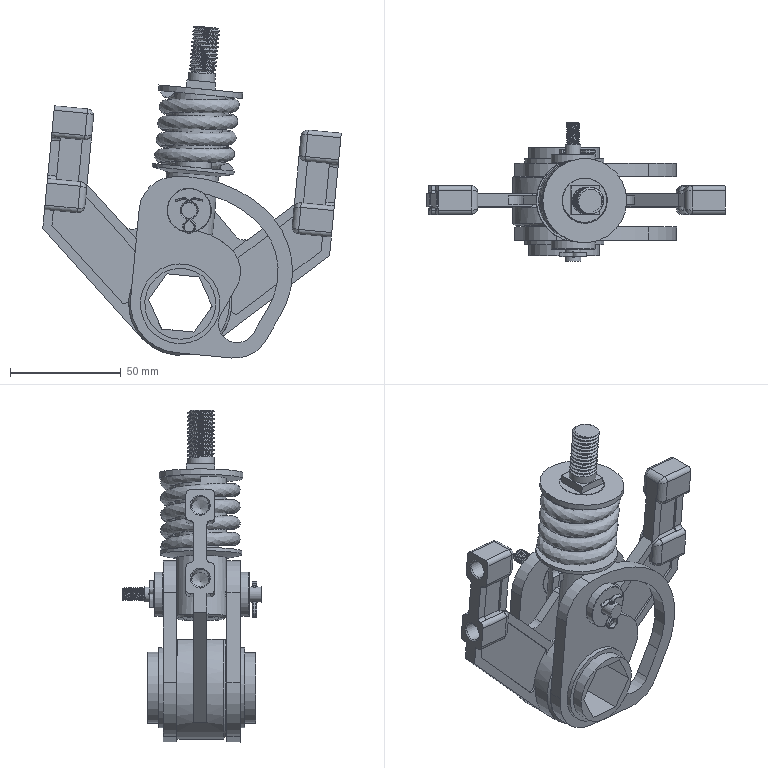Assembly | NX | mm | 14 component files | 14 solids | 384 faces | box 134.7 x 62.5 x 149.86 mm | volume 133468 mm3 | plane 178 | cylinder 147 | spline 30 | cone 23 | torus 6 | commonest cylinder face diameters 6 x25 4 x24 12 x12 7 x12 32 x8 3 x8 17 x6 10 x6
Bill of materials:
unnamed part 1 | 2 |  | Thick annular ring (spacer/washer-like) with a central through bore and small chamfers on the outer edges.
unnamed part 2 | 1 |  | Flat plate with a rounded, roughly D/teardrop outline, a large curved hook-shaped through slot, and a hexagonal feature with stepped cylindrical collars protruding on both faces.
unnamed part 3 | 1 |  | Flanged cylindrical sleeve with a thin wide flange, a through bore, a radial cross hole, and an axial slot running from the open end that ends in a rounded keyhole-like shape.
unnamed part 4 | 2 |  | Flat annular washer-like ring with a central through hole, thinner relative to its diameter than unnamed part 1, with small edge rounds or chamfers.
unnamed part 5 | 1 |  | Flanged plain bushing: cylindrical sleeve with a thin outer flange at one end, a through bore, an annular recess or counterbore on the flange face, and a chamfer at the other end.
unnamed part 6 | 1 |  | Bent strip or wire form clip: a closed circular eye, two parallel straight legs side by side, and leg ends that bend outward in opposite directions at an angle.
unnamed part 7 | 1 |  | Solid cylindrical pin with an external thread at one end and two radial cross holes, one near each end.
unnamed part 8 | 1 |  | Open helical coil spring of round wire with about four to five active turns and cut-off flat ends.
unnamed part 9 | 1 |  | Flat plate with a rounded, roughly D/teardrop outline, a large curved hook-shaped through slot, and a hexagonal feature with stepped cylindrical collars protruding on both faces.
unnamed part 10 | 1 |  | Stepped shaft with an external thread at one end, a thin collar/flange with an adjacent hexagonal section below the thread, a plain cylindrical shank, and a slotted opposite end with a cross hole/keyhole-shaped slot.
unnamed part 11 | 1 |  | Bent flat-strip clip: a closed circular eye, a long double-strip stem of two parallel legs, and two ends bent outward into short angled arms forming a T/Y shape.
unnamed part 12 | 1 |  | Bracket or fork made from a V/U-shaped plate with a central cylindrical ring boss and through bore, two angled arms ending in upright tabs with rectangular raised pads, and small countersunk holes in the tabs.
Mates:
1. touch align | tao 2 face | zhuanzhoutao 2 face
2. touch align | tao 1 face | zhuanzhoutao 1 face
3. touch align | tao 1 face | zhuanzhoutao 1 face
4. touch align | tongtao 2 face | zhuanzhoutao 2 face
5. touch align | tongtao 1 face | zhuanzhoutao 1 face
6. touch align | daozhu 1 face | dazhouzhicheng 1 face
7. touch align | xianweitao 1 face | daozhu 1 face
8. touch align | xiao 1 face | tongtao 1 face
9. touch align | dingtao 1 face | daozhu 1 face
10. touch align | yanhuang 1 face | dingtao 1 face